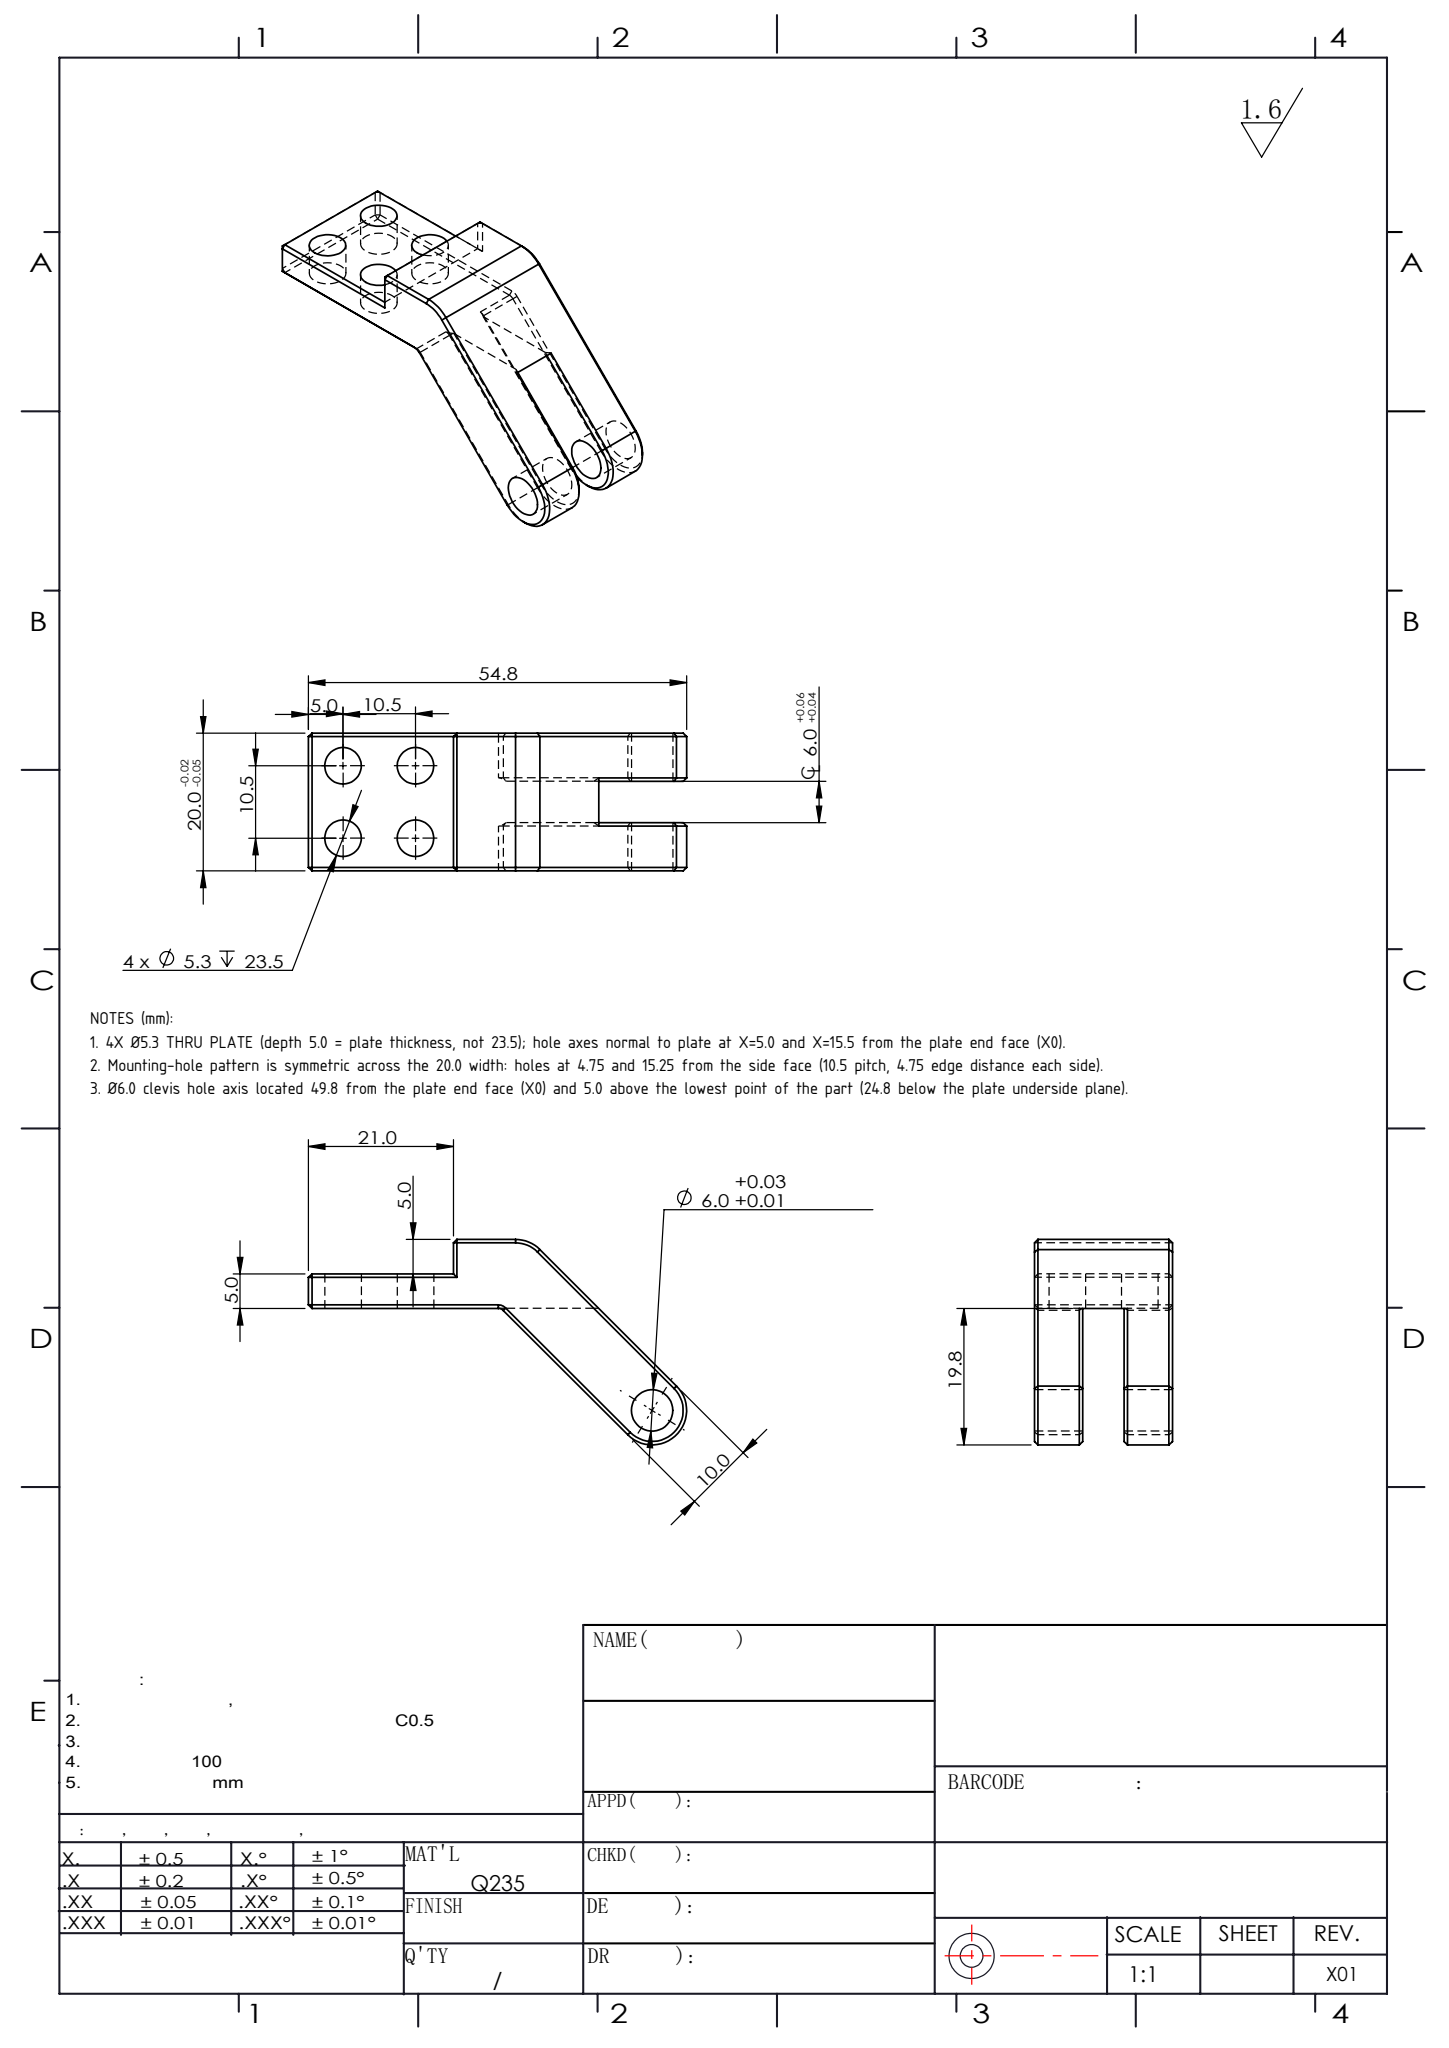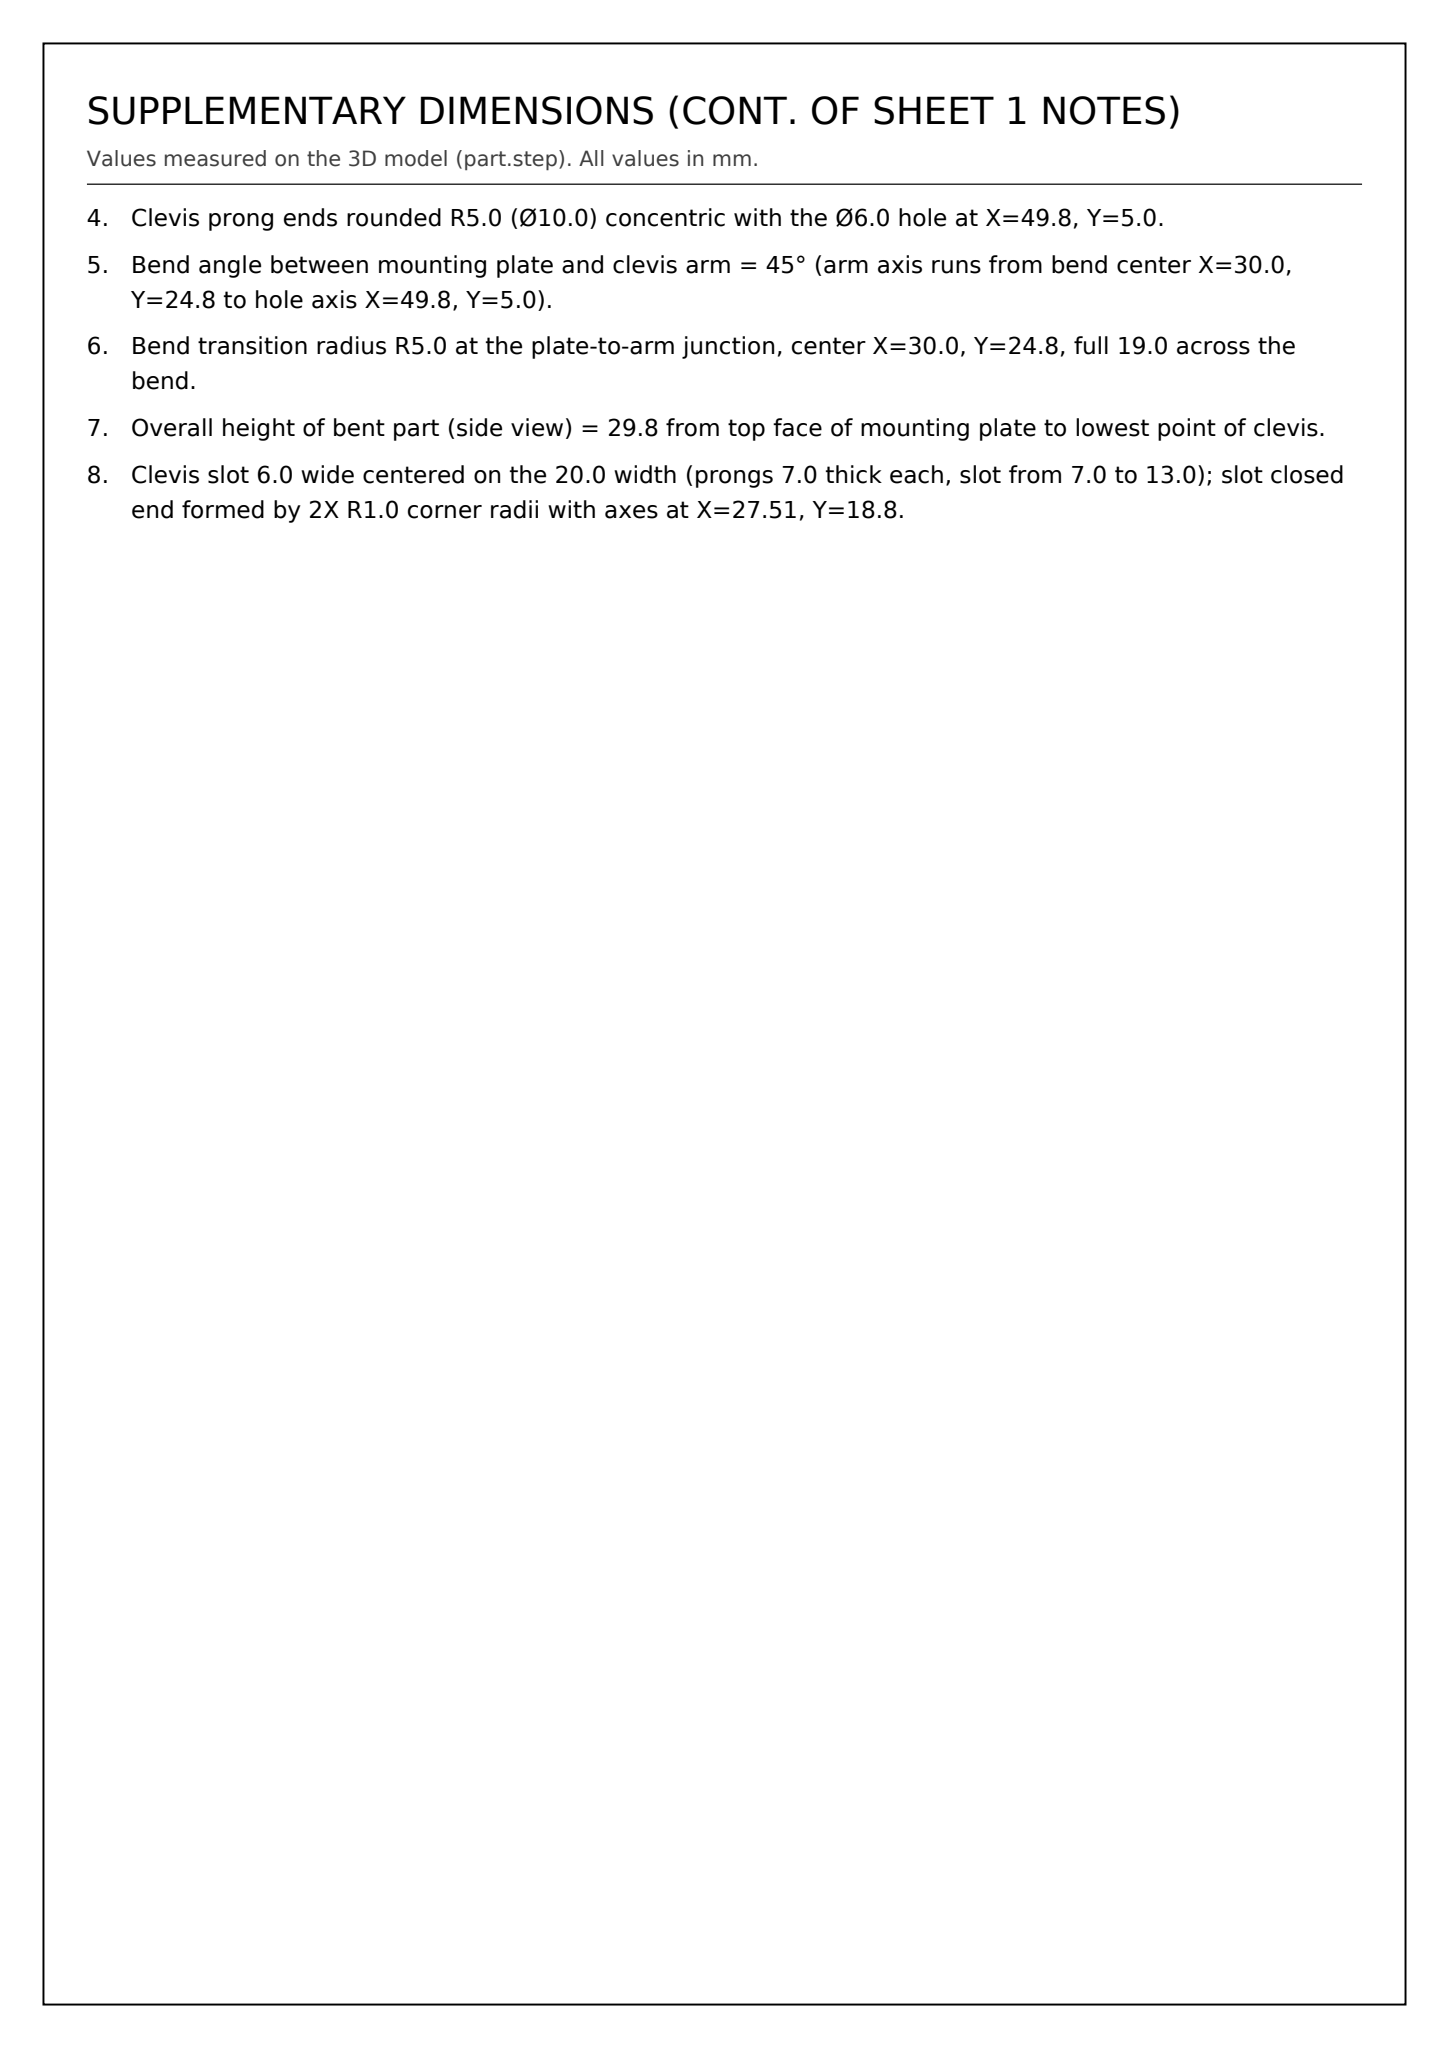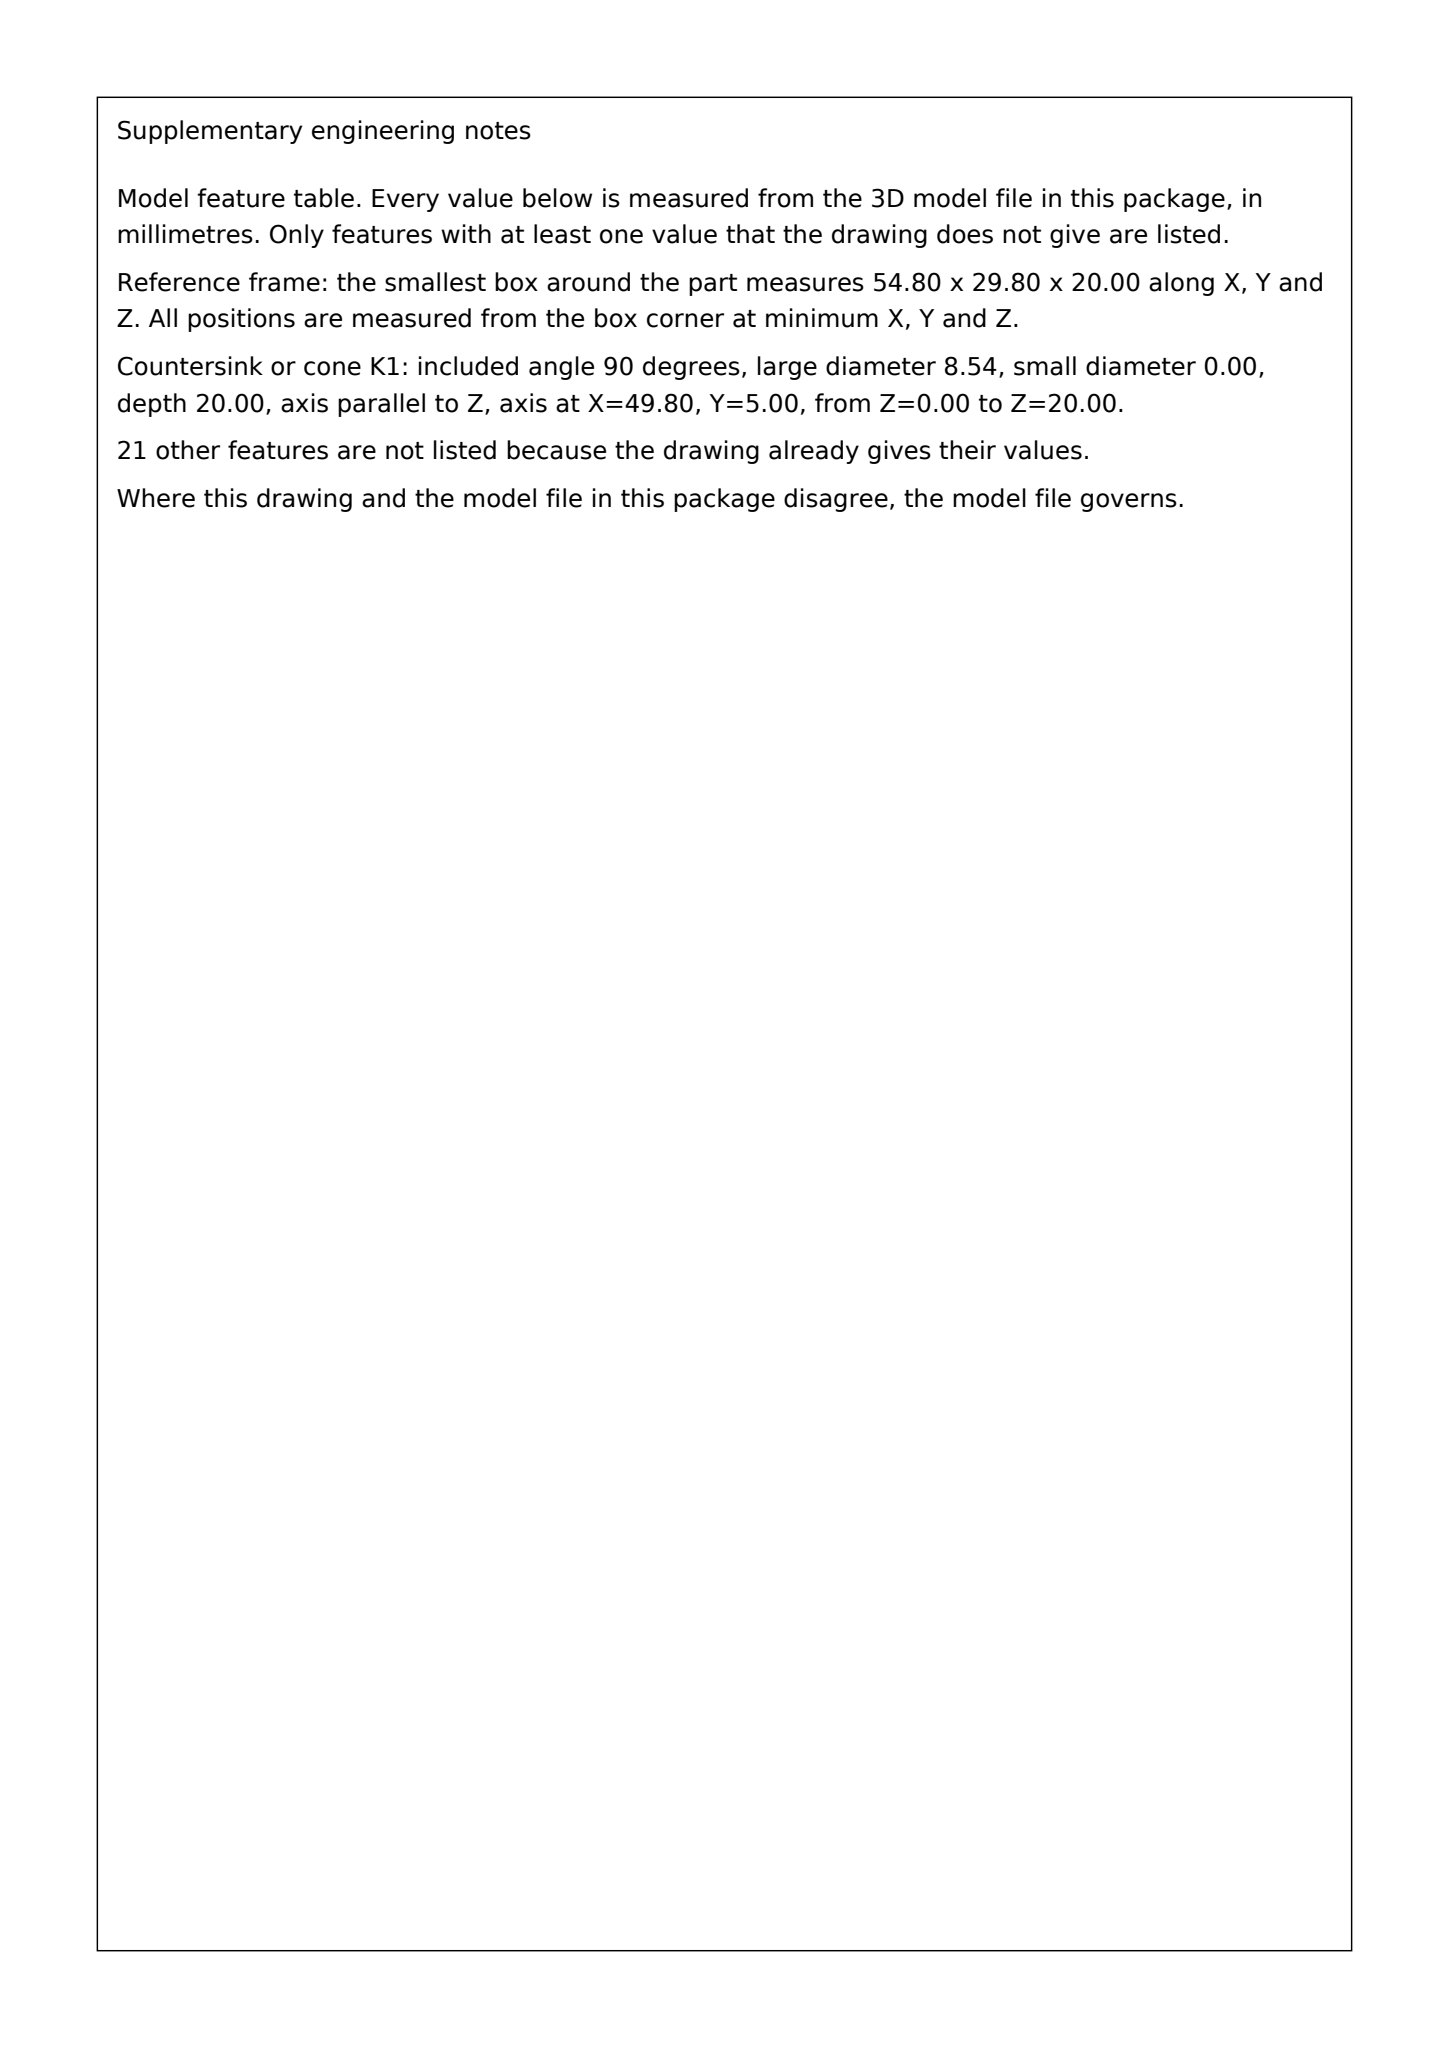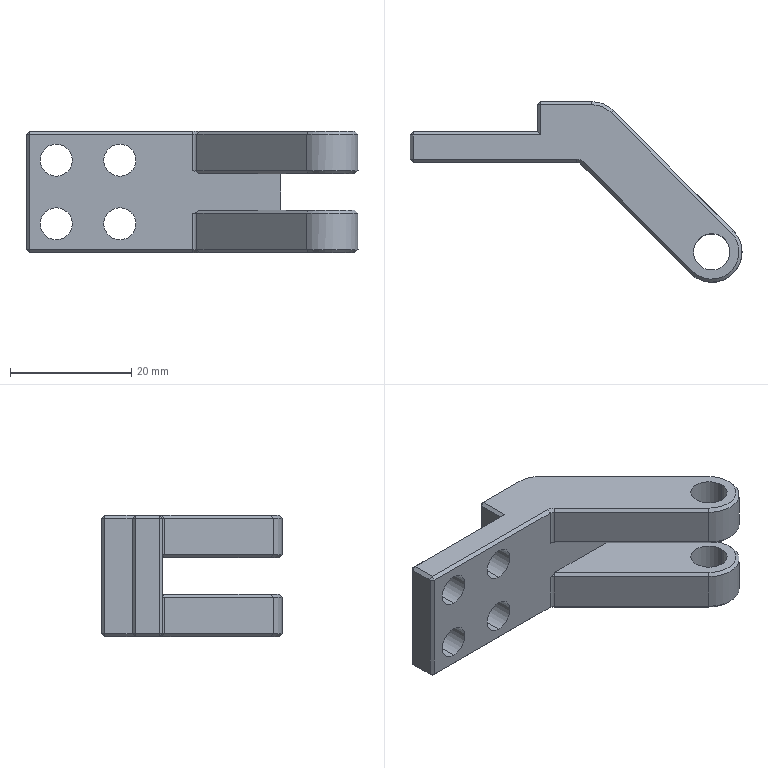Part | SolidWorks | mm | 1 solid | 68 faces | box 54.8 x 29.8 x 20 mm | volume 7890 mm3 | plane 39 | cylinder 17 | cone 12 | commonest cylinder face diameters 5.3 x8 6 x4 10 x3 2 x2
Drawing notes:
4X Ø5.3 THRU PLATE (depth 5.0 = plate thickness, not 23.5); hole axes normal to plate at X=5.0 and X=15.5 from the plate end face (X0). | from the solid: cylinders dia 5.3, axis y, pos x=5.0/15.5, length 5.0 (count 4)
Mounting-hole pattern is symmetric across the 20.0 width: holes at 4.75 and 15.25 from the side face (10.5 pitch, 4.75 edge distance each side). | from the solid: cylinders dia 5.3 at z=4.75 and z=15.25; bbox z = 20.0
Ø6.0 clevis hole axis located 49.8 from the plate end face (X0) and 5.0 above the lowest point of the part (24.8 below the plate underside plane). | from the solid: cylinders dia 6.0, axis z, pos (x=49.8, y=5.0), length 7.0
Clevis prong ends rounded R5.0 (Ø10.0) concentric with the Ø6.0 hole at X=49.8, Y=5.0. | from the solid: cylinders dia 10.0, axis z, pos (49.8, 5.0), length 6.0 (count 2)
Bend angle between mounting plate and clevis arm = 45° (arm axis runs from bend center X=30.0, Y=24.8 to hole axis X=49.8, Y=5.0). | from the solid: cylinder dia 10.0 pos (30.0, 24.8) and cylinders dia 6.0 pos (49.8, 5.0)
Bend transition radius R5.0 at the plate-to-arm junction, center X=30.0, Y=24.8, full 19.0 across the bend. | from the solid: cylinder dia 10.0, axis z, pos (30.0, 24.8), length 19.0
Overall height of bent part (side view) = 29.8 from top face of mounting plate to lowest point of clevis. | from the solid: bbox_xyz y = 29.799; plate faces at y=24.8 and y=29.8
Clevis slot 6.0 wide centered on the 20.0 width (prongs 7.0 thick each, slot from 7.0 to 13.0); slot closed end formed by 2X R1.0 corner radii with axes at X=27.51, Y=18.8. | from the solid: axis planes z=0/7/13/20; cylinders dia 2.0, axis z, pos (27.51, 18.8), length 6.0